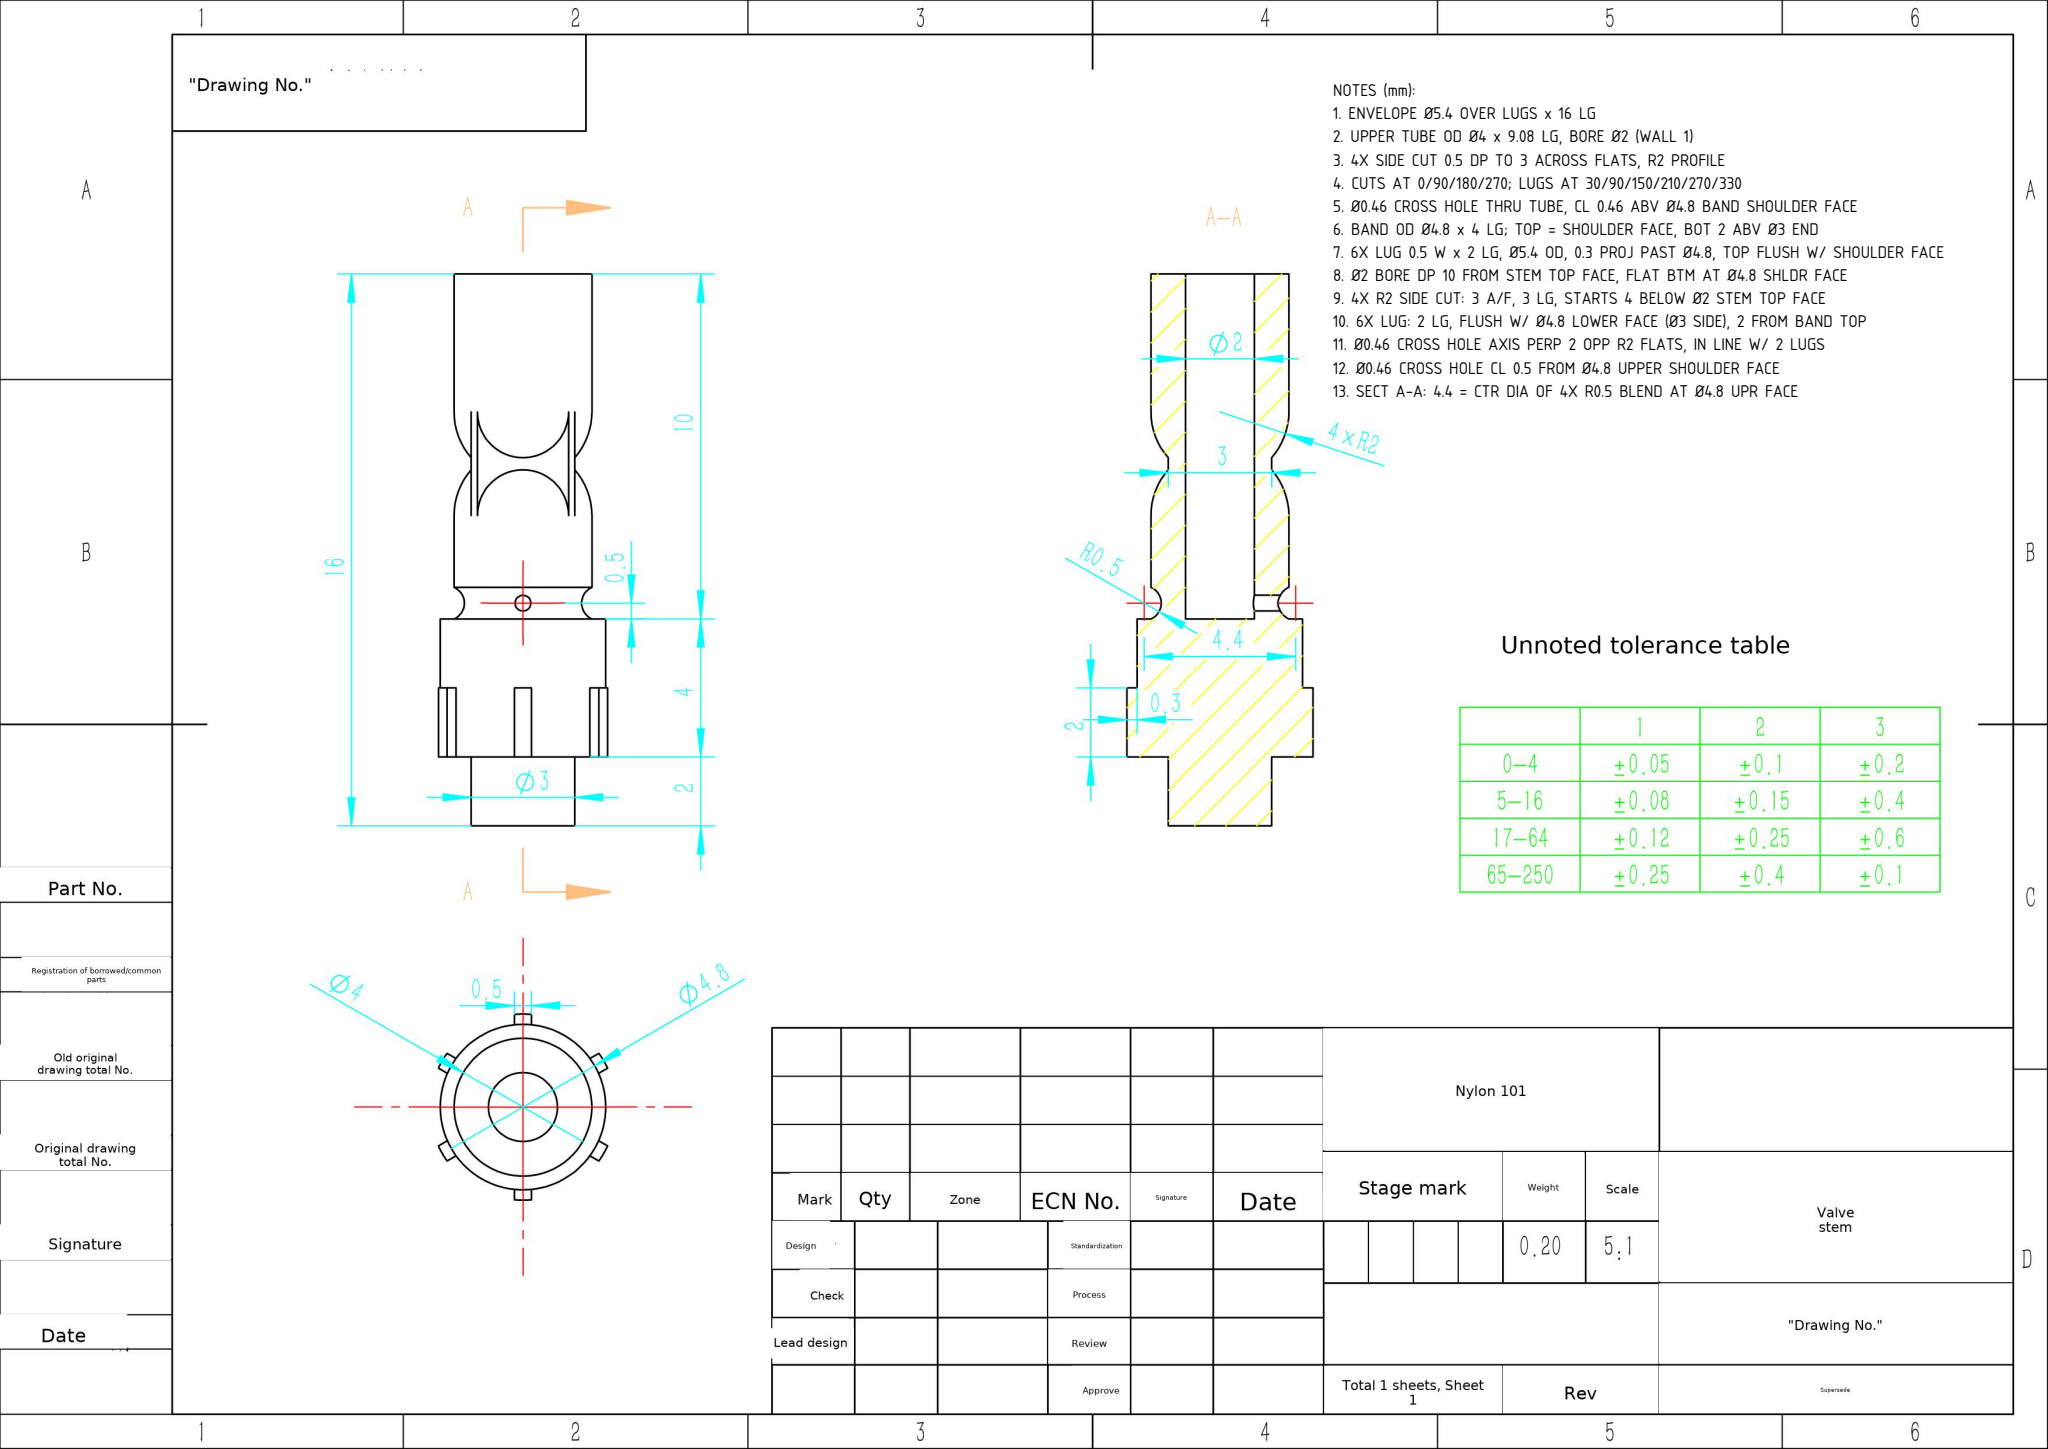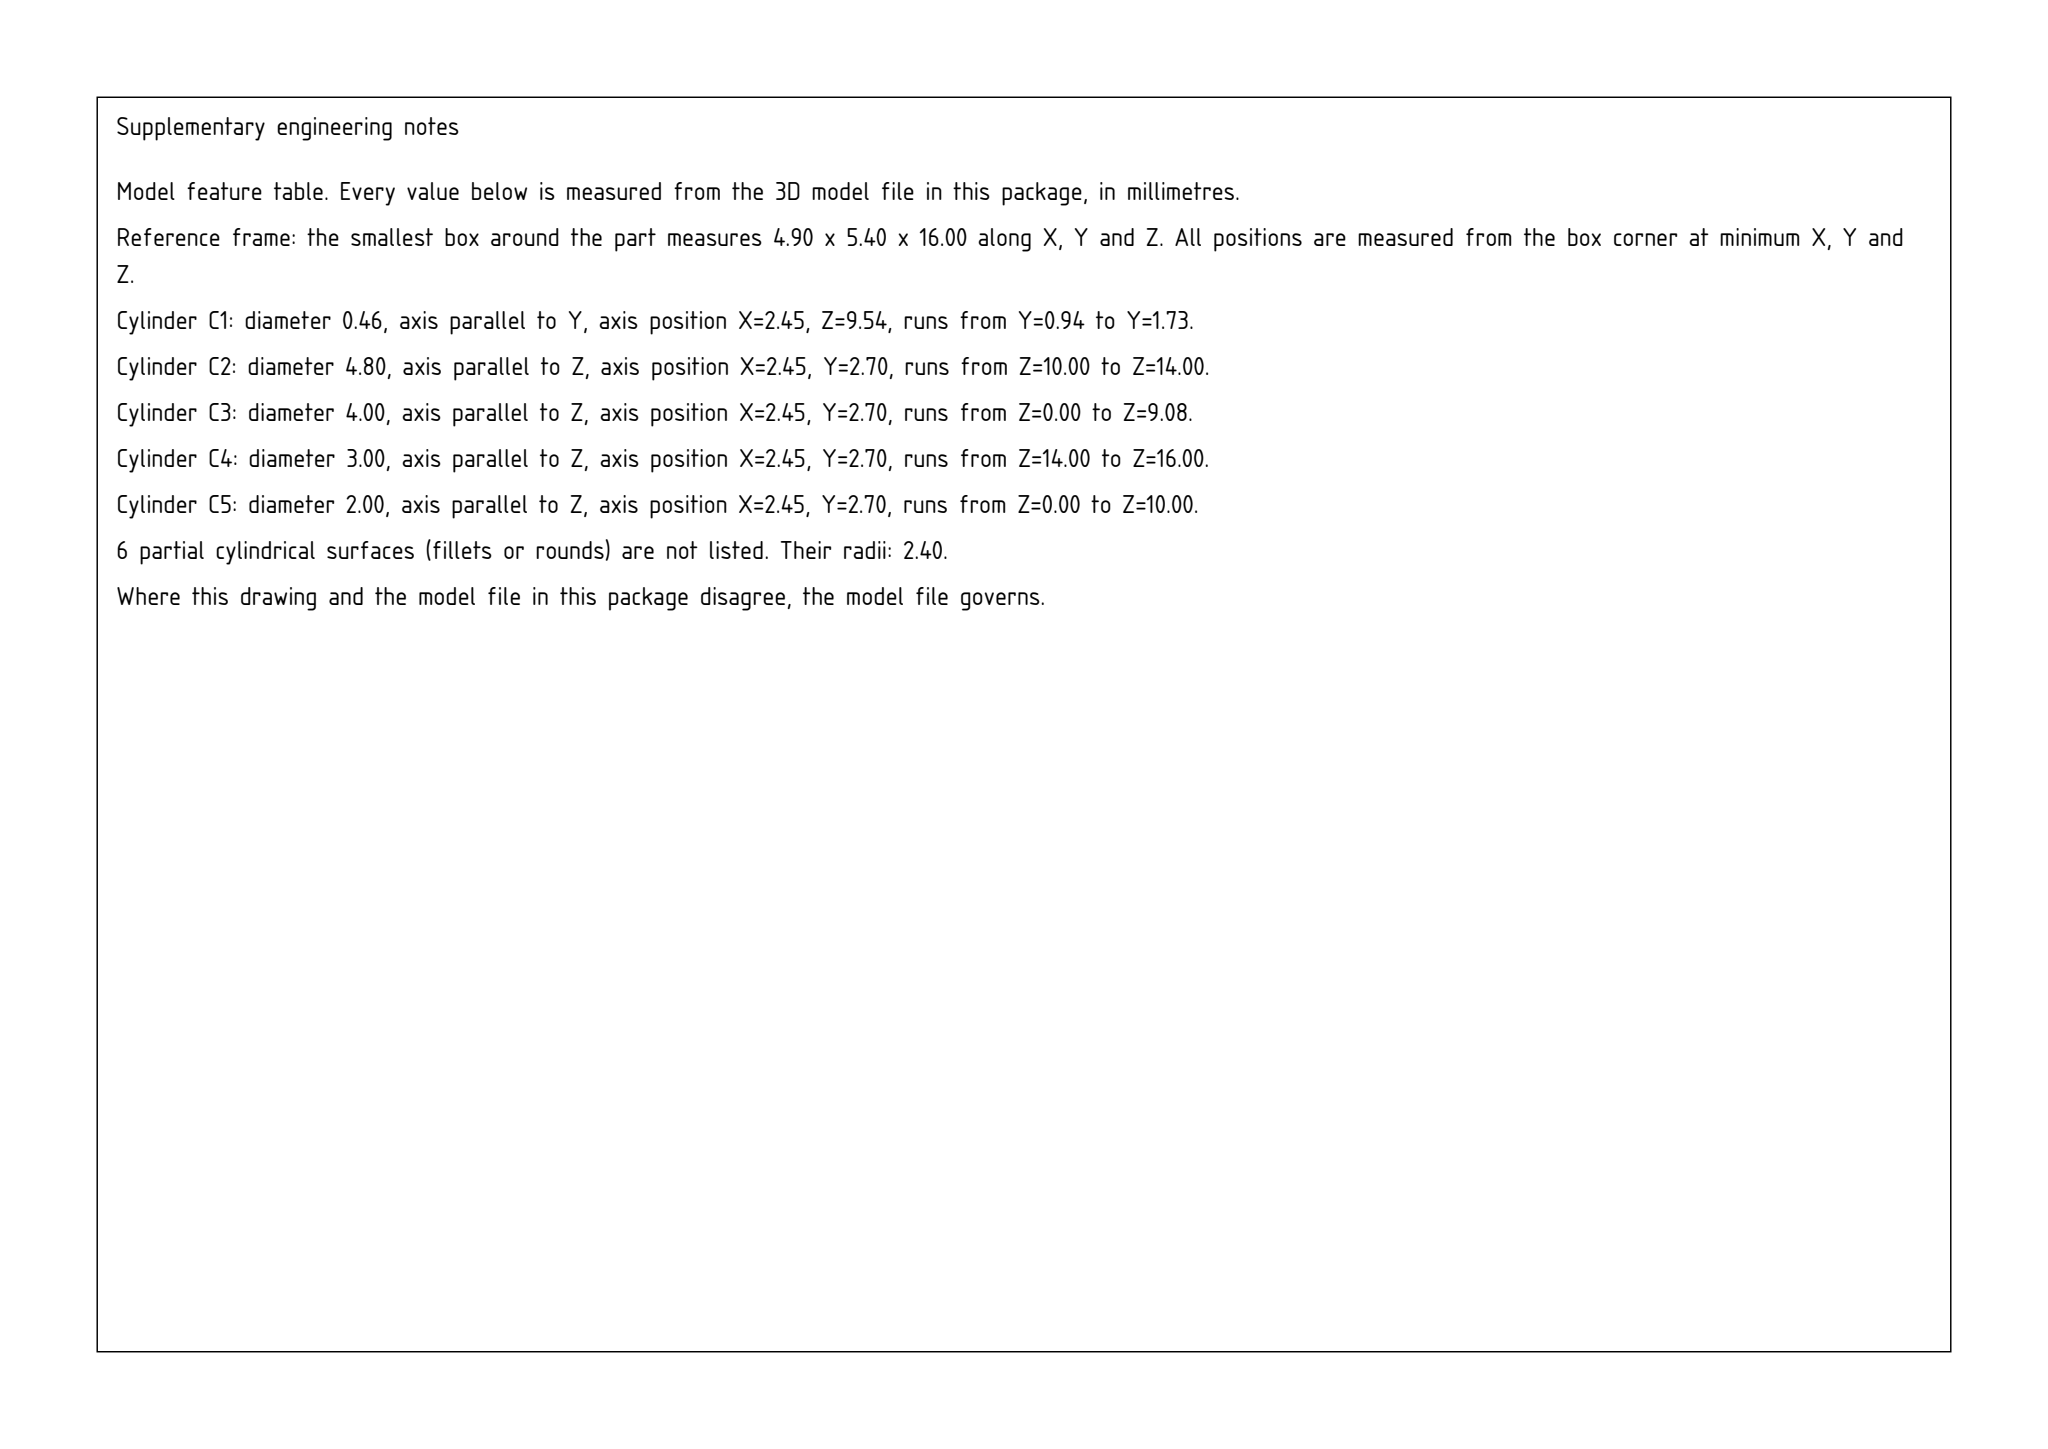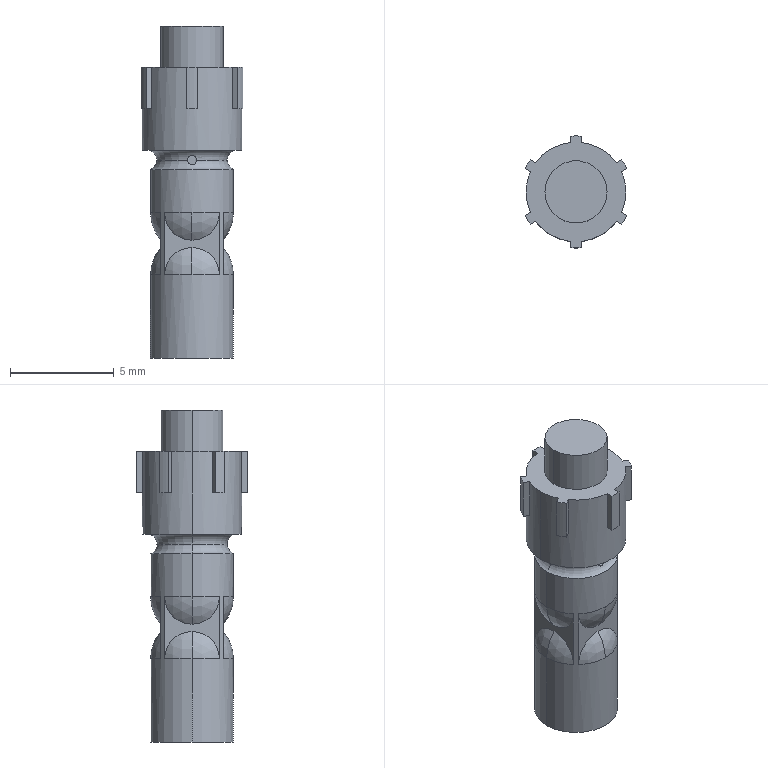Part | SolidWorks | mm | 1 solid | 63 faces | box 4.9 x 5.4 x 16 mm | volume 175 mm3 | plane 27 | sphere 16 | cylinder 16 | torus 4 | commonest cylinder face diameters 4.8 x8 0.46 x2 2 x2 3 x2 4 x2
Drawing notes:
ENVELOPE Ø5.4 OVER LUGS x 16 LG | from the solid: bbox 4.904 x 5.4 x 16.0; lugs project to Ø5.4
UPPER TUBE OD Ø4 x 9.08 LG, BORE Ø2 (WALL 1) | from the solid: cyl [4.0,z,(2.45,2.7),9.08] over coaxial bore cyl [2.0,z,(2.45,2.7),10.0]
4X SIDE CUT 0.5 DP TO 3 ACROSS FLATS, R2 PROFILE | from the solid: planes x=0.95/3.95, y=1.2/4.2 = 1.5 from axis (3 across flats) on Ø4; 4 x R2
CUTS AT 0/90/180/270; LUGS AT 30/90/150/210/270/330 | from the solid: flats normal to X and Y; 6 lug cyls offset 0.3 at 30/90/150/210/270/330
Ø0.46 CROSS HOLE THRU TUBE, CL 0.46 ABV Ø4.8 BAND SHOULDER FACE | from the solid: 2 cyls dia 0.46 axis y at (x=2.45, z=9.54) thru Ø4 wall; shoulder face plane z=10
BAND OD Ø4.8 x 4 LG; TOP = SHOULDER FACE, BOT 2 ABV Ø3 END | from the solid: Ø4.8 cyl len 4 at axis (2.45,2.7), z=10 to 14; Ø3 cyl len 2 z=14 to 16
6X LUG 0.5 W x 2 LG, Ø5.4 OD, 0.3 PROJ PAST Ø4.8, TOP FLUSH W/ SHOULDER FACE | from the solid: Ø4.8 lug cyls offset 0.3 from axis, len 2.0 z=10 to 12 (6 planes at z=12); bbox y=5.4
Ø2 BORE DP 10 FROM STEM TOP FACE, FLAT BTM AT Ø4.8 SHLDR FACE | from the solid: cylinder dia 2.0 axis z at (2.45,2.7), length 10.0, running from top face plane z=0 to z=10, which is the Ø4.8 band top face plane (z=10); Ø4 stem face spans z=0..9.08, band 10..14, Ø3 boss 14..16
4X R2 SIDE CUT: 3 A/F, 3 LG, STARTS 4 BELOW Ø2 STEM TOP FACE | from the solid: Flat planes x=1.0 & x=4.0 and y=1.2 & y=4.2 (3 across flats, axis at x2.5,y2.7), z extent 4.0-7.0; part top face z=0
6X LUG: 2 LG, FLUSH W/ Ø4.8 LOWER FACE (Ø3 SIDE), 2 FROM BAND TOP | from the solid: Lug faces/inclined flanks z=12.0 to 14.0, size z=2.0; Ø4.8 band z=10.0-14.0, Ø3 boss z=14.0-16.0
Ø0.46 CROSS HOLE AXIS PERP 2 OPP R2 FLATS, IN LINE W/ 2 LUGS | from the solid: Hole dia 0.46 axis = Y at x2.5,z9.5; y-normal flats at y=1.2/4.2; lugs at 90°/270° (x2.2-2.7, y0-0.3 & y5.1-5.4)
Ø0.46 CROSS HOLE CL 0.5 FROM Ø4.8 UPPER SHOULDER FACE | from the solid: Hole axis at z=9.5; Ø4.8 band upper face plane z=10.0
SECT A-A: 4.4 = CTR DIA OF 4X R0.5 BLEND AT Ø4.8 UPR FACE | from the solid: tori minor_r 0.5, major_r 2.2 (x4) => center circle dia 4.4, at Ø4-to-Ø4.8 transition z=9.1-10.0
build123d program:
from build123d import *

# Parameters (mm, degrees)
SKETCH1_R                  = 2
BOSS_EXTRUDE1_DEPTH        = 10
SKETCH3_R                  = 0.5
SKETCH2_R                  = 2.4
BOSS_EXTRUDE2_DEPTH        = 4
SKETCH4_R                  = 1.5
BOSS_EXTRUDE3_DEPTH        = 2
CUT_EXTRUDE1_START         = -6
SKETCH5_R                  = 1
CUT_EXTRUDE1_DEPTH         = 11.356
SKETCH6_R                  = 0.23
CUT_EXTRUDE2_DEPTH         = 17.356
SKETCH7_W                  = 0.5
SKETCH7_H                  = 3
CUT_EXTRUDE6_DEPTH         = 17.356
CIRPATTERN1_COUNT          = 2
CIRPATTERN1_ANGLE          = 90
CIRPATTERN2_COUNT          = 4
BOSS_EXTRUDE4_REACH        = 18.656
BOSS_EXTRUDE4_START_RADIUS = 2.4
BOSS_EXTRUDE4_END_RADIUS   = 2.4
SKETCH10_W                 = 0.5
SKETCH10_H                 = 2
CIRPATTERN3_COUNT          = 6


with BuildPart() as part:
    # Sketch1 → Boss-Extrude1 (new body)
    with BuildSketch(Plane.XY):
        Circle(SKETCH1_R)
    extrude(amount=BOSS_EXTRUDE1_DEPTH)

    # Sketch3 → Cut-Revolve1 (revolve, cut)
    with BuildSketch(Plane(origin=(0, 0, 0), x_dir=(1, 0, 0), z_dir=(0, 1, 0)), mode=Mode.PRIVATE) as cut_revolve1_sk:
        with Locations((-2.2, -9.542)):
            Circle(SKETCH3_R)
    revolve(cut_revolve1_sk.sketch.rotate(Axis((0, 0, 10), (0, 0, -1)), 180), axis=Axis((0, 0, 10), (0, 0, -1)), mode=Mode.SUBTRACT)

    # Sketch2 → Boss-Extrude2 (add)
    with BuildSketch(Plane.XY.offset(10)):
        Circle(SKETCH2_R)
    extrude(amount=BOSS_EXTRUDE2_DEPTH)

    # Sketch4 → Boss-Extrude3 (add)
    with BuildSketch(Plane.XY.offset(14)):
        Circle(SKETCH4_R)
    extrude(amount=BOSS_EXTRUDE3_DEPTH)

    # Sketch5 → Cut-Extrude1 (cut, through all)
    with BuildSketch(Plane.XY.offset(16).offset(CUT_EXTRUDE1_START)):
        Circle(SKETCH5_R)
    extrude(amount=-CUT_EXTRUDE1_DEPTH, mode=Mode.SUBTRACT)

    # Sketch6 → Cut-Extrude2 (cut, through all)
    with BuildSketch(Plane(origin=(0, 0, 0), x_dir=(1, 0, 0), z_dir=(0, 1, 0))):
        with Locations(Location((0, -9.542, 0), (0, 0, 270))):
            Circle(SKETCH6_R)
    extrude(amount=-CUT_EXTRUDE2_DEPTH, mode=Mode.SUBTRACT)

    # Sketch7 → Cut-Extrude6 (cut, symmetric)
    with BuildSketch(Plane(origin=(0, 0, 0), x_dir=(1, 0, 0), z_dir=(0, 1, 0))):
        with Locations((1.75, -5.5)):
            Rectangle(SKETCH7_W, SKETCH7_H)
        with Locations((-1.75, -5.5)):
            Rectangle(SKETCH7_W, SKETCH7_H)
    cut_extrude6 = extrude(amount=CUT_EXTRUDE6_DEPTH, both=True, mode=Mode.SUBTRACT)

    # CirPattern1: Cut-Extrude6 ×2 about axis
    cirpattern1_axis = Axis((0, 0, 10), (0, 0, -1))
    for i in range(1, CIRPATTERN1_COUNT):
        add(cut_extrude6.rotate(cirpattern1_axis, i * CIRPATTERN1_ANGLE / (CIRPATTERN1_COUNT - 1)), mode=Mode.SUBTRACT)

    # Sketch8 → Revolve2 (revolve)
    with BuildSketch(Plane(origin=(0, 0, 0), x_dir=(0, 0, -1), z_dir=(1, 0, 0))):
        with BuildLine():
            Line((-4, -1.5), (-5.323, -1.5))
            ThreePointArc((-5.323, -1.5), (-4.707, -1.871), (-4, -2))
            Line((-4, -2), (-4, -1.5))
        make_face()
    revolve2 = revolve(axis=Axis((0, -1.5, 4), (0, -1, 0)))

    # Mirror1: Revolve2 across plane
    add(revolve2.mirror(Plane.XY.offset(5.5)))

    # CirPattern2: Revolve2 ×4 about axis
    cirpattern2_axis = Axis((0, 0, 10), (0, 0, -1))
    for i in range(1, CIRPATTERN2_COUNT):
        add(revolve2.rotate(cirpattern2_axis, i * 360 / CIRPATTERN2_COUNT))

    # CirPattern2 copy 1 sketch → CirPattern2 copy 1 (revolve)
    with BuildSketch(Plane(origin=(0, 0, 11), x_dir=(0, 0, 1), z_dir=(0, -1, 0))):
        with BuildLine():
            Line((-4, 1.5), (-5.323, 1.5))
            ThreePointArc((-5.323, 1.5), (-4.707, 1.871), (-4, 2))
            Line((-4, 2), (-4, 1.5))
        make_face()
    revolve(axis=Axis((-1.5, 0, 7), (1, 0, 0)))

    # CirPattern2 copy 2 sketch → CirPattern2 copy 2 (revolve)
    with BuildSketch(Plane(origin=(0, 0, 11), x_dir=(0, 0, 1), z_dir=(-1, 0, 0))):
        with BuildLine():
            Line((-4, 1.5), (-5.323, 1.5))
            ThreePointArc((-5.323, 1.5), (-4.707, 1.871), (-4, 2))
            Line((-4, 2), (-4, 1.5))
        make_face()
    revolve(axis=Axis((0, 1.5, 7), (0, -1, 0)))

    # CirPattern2 copy 3 sketch → CirPattern2 copy 3 (revolve)
    with BuildSketch(Plane(origin=(0, 0, 11), x_dir=(0, 0, 1), z_dir=(0, 1, 0))):
        with BuildLine():
            Line((-4, 1.5), (-5.323, 1.5))
            ThreePointArc((-5.323, 1.5), (-4.707, 1.871), (-4, 2))
            Line((-4, 2), (-4, 1.5))
        make_face()
    revolve(axis=Axis((1.5, 0, 7), (-1, 0, 0)))

    # Boss-Extrude4: from a cylinder face, 18.656 long prism both ways, kept between that surface and its translate by the depth
    boss_extrude4_start = Plane(origin=(0, 0, 13), z_dir=(0, 0, -1)) * Cylinder(BOSS_EXTRUDE4_START_RADIUS, 43.112, mode=Mode.PRIVATE)
    boss_extrude4_end = Plane(origin=(0, 0.3, 13), z_dir=(0, 0, -1)) * Cylinder(BOSS_EXTRUDE4_END_RADIUS, 43.112, mode=Mode.PRIVATE)
    # Sketch10 → Boss-Extrude4 (add, from a surface)
    with BuildSketch(Plane(origin=(0, 0, 0), x_dir=(1, 0, 0), z_dir=(0, 1, 0)), mode=Mode.PRIVATE) as boss_extrude4_sk1:
        with Locations((0, -13)):
            Rectangle(SKETCH10_W, SKETCH10_H)
    boss_extrude4_tool1 = extrude(boss_extrude4_sk1.sketch, amount=BOSS_EXTRUDE4_REACH, both=True, mode=Mode.PRIVATE)
    boss_extrude4 = ((boss_extrude4_tool1 - boss_extrude4_start) & boss_extrude4_end).solids().sort_by_distance((0, 2.537, 13))[0]
    add(boss_extrude4)

    # CirPattern3: Boss-Extrude4 ×6 about axis
    cirpattern3_axis = Axis((0, 0, 0), (0, 0, 1))
    for i in range(1, CIRPATTERN3_COUNT):
        add(boss_extrude4.rotate(cirpattern3_axis, i * 360 / CIRPATTERN3_COUNT))


solid = part.part